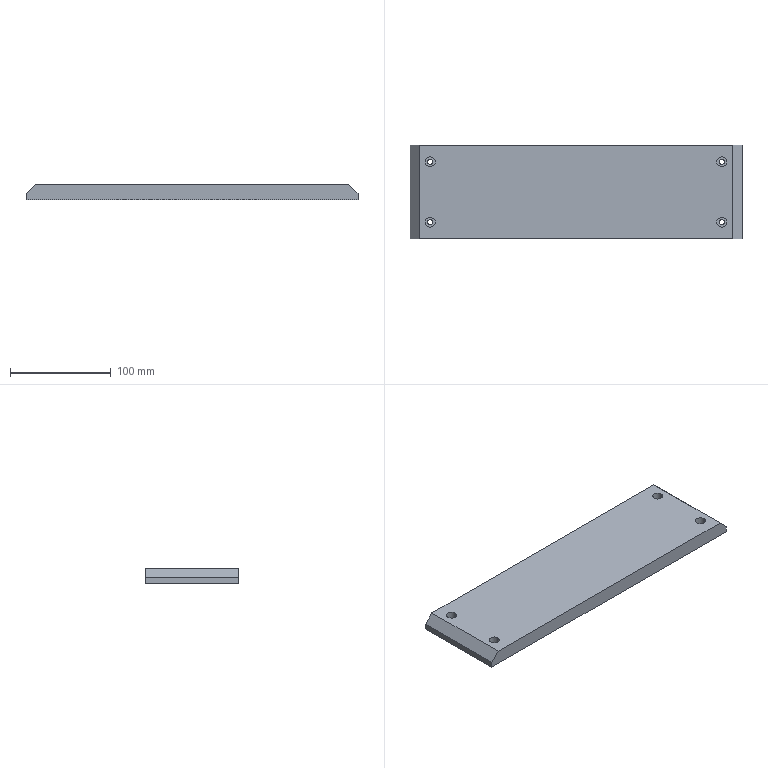CAM job | Mastercam | mm | 3 operations | part box 330 x 93 x 15
1. Surface Finish Flowline | 9 - 8 圆鼻铣刀
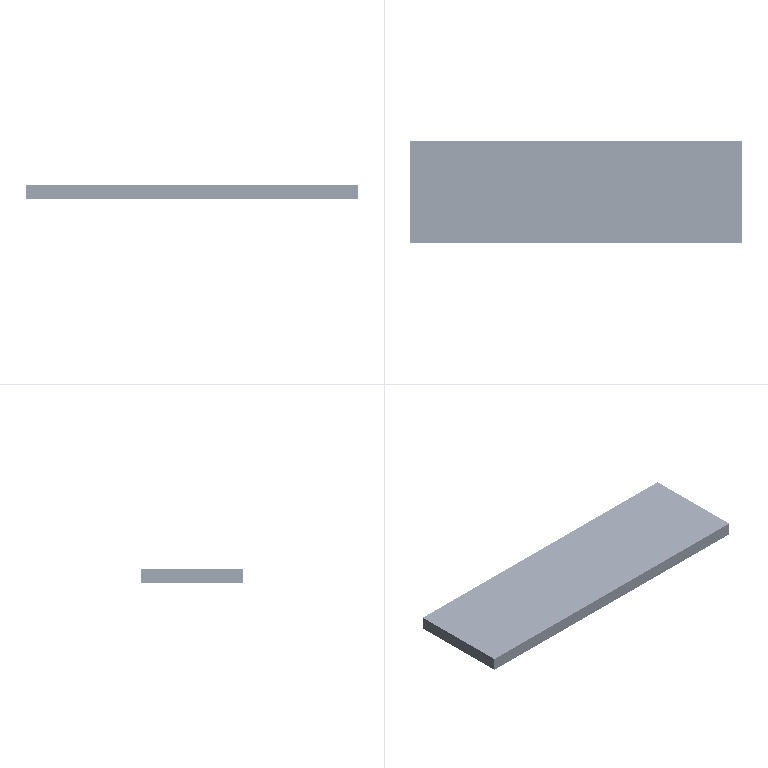2. Contour (Ramp) | 6 - 6 平铣刀
3. Drill/Counterbore | 7 - 4 倒角刀